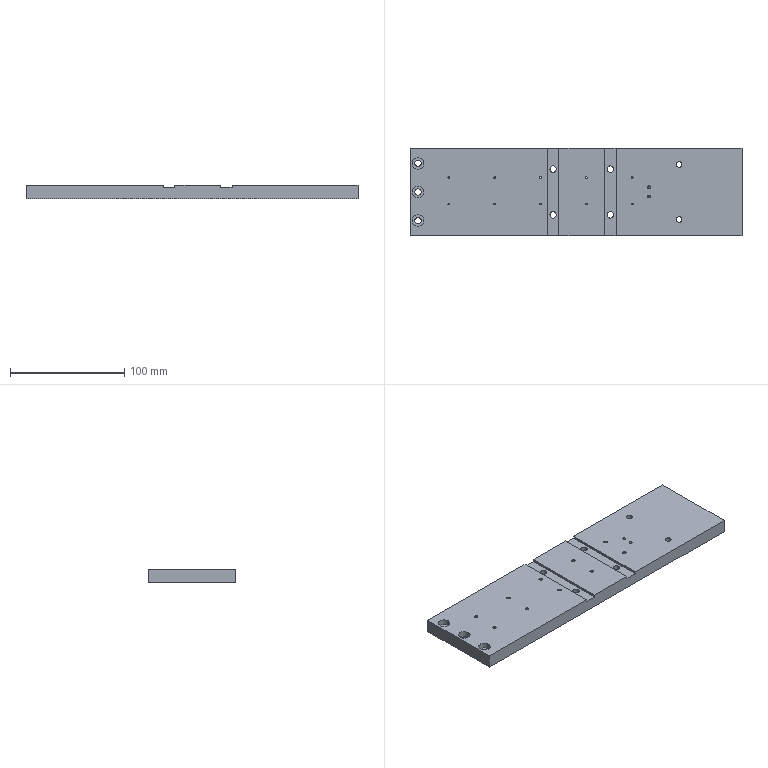Component | SolidWorks | ServoVerticalBasePlate-2-1 | 1 solid | 113 faces | box 290 x 76 x 12 mm | volume 255552 mm3 | cylinder 62 | cone 30 | plane 21 | commonest cylinder face diameters 3.3 x20 10 x14 5.5 x14 4.2 x6 2.5 x4 5 x4 | material Plain Carbon Steel
build123d program:
from build123d import *

# Parameters (mm, degrees)
SKETCH1_W                                            = 290
SKETCH1_H                                            = 76
BOSS_EXTRUDE1_DEPTH                                  = 12
CYLINDRICAL_COUNTERSUNK_HOLE_FOR_M5_SOCK_D           = 5.5
CYLINDRICAL_COUNTERSUNK_HOLE_FOR_M5_SOCK_CBORE_D     = 10
CYLINDRICAL_COUNTERSUNK_HOLE_FOR_M5_SOCK_CBORE_DEPTH = 5
M5_TAPPED_HOLE1_D                                    = 4.2
M5_TAPPED_HOLE1_DEPTH                                = 14
M5_TAPPED_HOLE1_TIP                                  = 1.262
M6_TAPPED_HOLE1_D                                    = 5
M6_TAPPED_HOLE1_DEPTH                                = 17
M6_TAPPED_HOLE1_TIP                                  = 1.502
CYLINDRICAL_COUNTERSUNK_HOLE_FOR_M5_2_D              = 5.5
CYLINDRICAL_COUNTERSUNK_HOLE_FOR_M5_2_CBORE_D        = 10
CYLINDRICAL_COUNTERSUNK_HOLE_FOR_M5_2_CBORE_DEPTH    = 5
SKETCH12_W                                           = 10
SKETCH12_H                                           = 2
CUT_EXTRUDE1_DEPTH                                   = 80
M4_TAPPED_HOLE1_D                                    = 3.3
M4_TAPPED_HOLE1_DEPTH                                = 11.5
M4_TAPPED_HOLE1_TIP                                  = 0.9914
M3_TAPPED_HOLE1_D                                    = 2.5
M3_TAPPED_HOLE1_DEPTH                                = 8.5
M3_TAPPED_HOLE1_TIP                                  = 0.7511


with BuildPart() as part:
    # Sketch1 → Boss-Extrude1 (new body)
    with BuildSketch(Plane.XY):
        with Locations((145, 38)):
            Rectangle(SKETCH1_W, SKETCH1_H)
    extrude(amount=BOSS_EXTRUDE1_DEPTH)

    # Cylindrical Countersunk Hole for M5 Sock (through all)
    with Locations(Plane.XY.offset(12)):
        with Locations((7, 63), (7, 38), (7, 13)):
            CounterBoreHole(CYLINDRICAL_COUNTERSUNK_HOLE_FOR_M5_SOCK_D / 2, CYLINDRICAL_COUNTERSUNK_HOLE_FOR_M5_SOCK_CBORE_D / 2, CYLINDRICAL_COUNTERSUNK_HOLE_FOR_M5_SOCK_CBORE_DEPTH)

    # M5 Tapped Hole1
    with Locations(Plane(origin=(290, 0, 0), x_dir=(0, 0, -1), z_dir=(1, 0, 0))):
        with Locations((-6, 66), (-6, 38), (-6, 10)):
            Hole(M5_TAPPED_HOLE1_D / 2, depth=M5_TAPPED_HOLE1_DEPTH)
            with Locations((0, 0, -(M5_TAPPED_HOLE1_DEPTH + M5_TAPPED_HOLE1_TIP / 2))):  # 118° drill point
                Cone(0, M5_TAPPED_HOLE1_D / 2, M5_TAPPED_HOLE1_TIP, mode=Mode.SUBTRACT)

    # M6 Tapped Hole1
    with Locations(Plane(origin=(0, 0, 0), x_dir=(-1, 0, 0), z_dir=(0, 0, -1))):
        with Locations((-235, 14), (-235, 62)):
            Hole(M6_TAPPED_HOLE1_D / 2, depth=M6_TAPPED_HOLE1_DEPTH)
            with Locations((0, 0, -(M6_TAPPED_HOLE1_DEPTH + M6_TAPPED_HOLE1_TIP / 2))):  # 118° drill point
                Cone(0, M6_TAPPED_HOLE1_D / 2, M6_TAPPED_HOLE1_TIP, mode=Mode.SUBTRACT)

    # Cylindrical Countersunk Hole for M5  2 (through all)
    with Locations(Plane(origin=(0, 0, 0), x_dir=(-1, 0, 0), z_dir=(0, 0, -1))):
        with Locations((-175, 58), (-125, 58), (-125, 18), (-175, 18)):
            CounterBoreHole(CYLINDRICAL_COUNTERSUNK_HOLE_FOR_M5_2_D / 2, CYLINDRICAL_COUNTERSUNK_HOLE_FOR_M5_2_CBORE_D / 2, CYLINDRICAL_COUNTERSUNK_HOLE_FOR_M5_2_CBORE_DEPTH)

    # Sketch12 → Cut-Extrude1 (cut)
    with BuildSketch(Plane(origin=(0, 76, 0), x_dir=(1, 0, 0), z_dir=(0, 1, 0))):
        with Locations((175, -11)):
            Rectangle(SKETCH12_W, SKETCH12_H)
        with Locations((125, -11)):
            Rectangle(SKETCH12_W, SKETCH12_H)
    extrude(amount=-CUT_EXTRUDE1_DEPTH, mode=Mode.SUBTRACT)

    # M4 Tapped Hole1
    with Locations(Plane(origin=(0, 0, 0), x_dir=(-1, 0, 0), z_dir=(0, 0, -1))):
        with Locations((-194, 50.5), (-194, 27.5), (-154, 50.5), (-154, 27.5), (-114, 50.5), (-114, 27.5), (-74, 27.5), (-74, 50.5), (-34, 50.5), (-34, 27.5)):
            Hole(M4_TAPPED_HOLE1_D / 2, depth=M4_TAPPED_HOLE1_DEPTH)
            with Locations((0, 0, -(M4_TAPPED_HOLE1_DEPTH + M4_TAPPED_HOLE1_TIP / 2))):  # 118° drill point
                Cone(0, M4_TAPPED_HOLE1_D / 2, M4_TAPPED_HOLE1_TIP, mode=Mode.SUBTRACT)

    # M3 Tapped Hole1
    with Locations(Plane.XY.offset(12)):
        with Locations((208.75, 34), (208.75, 42)):
            Hole(M3_TAPPED_HOLE1_D / 2, depth=M3_TAPPED_HOLE1_DEPTH)
            with Locations((0, 0, -(M3_TAPPED_HOLE1_DEPTH + M3_TAPPED_HOLE1_TIP / 2))):  # 118° drill point
                Cone(0, M3_TAPPED_HOLE1_D / 2, M3_TAPPED_HOLE1_TIP, mode=Mode.SUBTRACT)


solid = part.part

# Placed as in the assembly
solid = solid.moved(Location((-195.522, -18.055, 36.551), (0, 0, 0)))